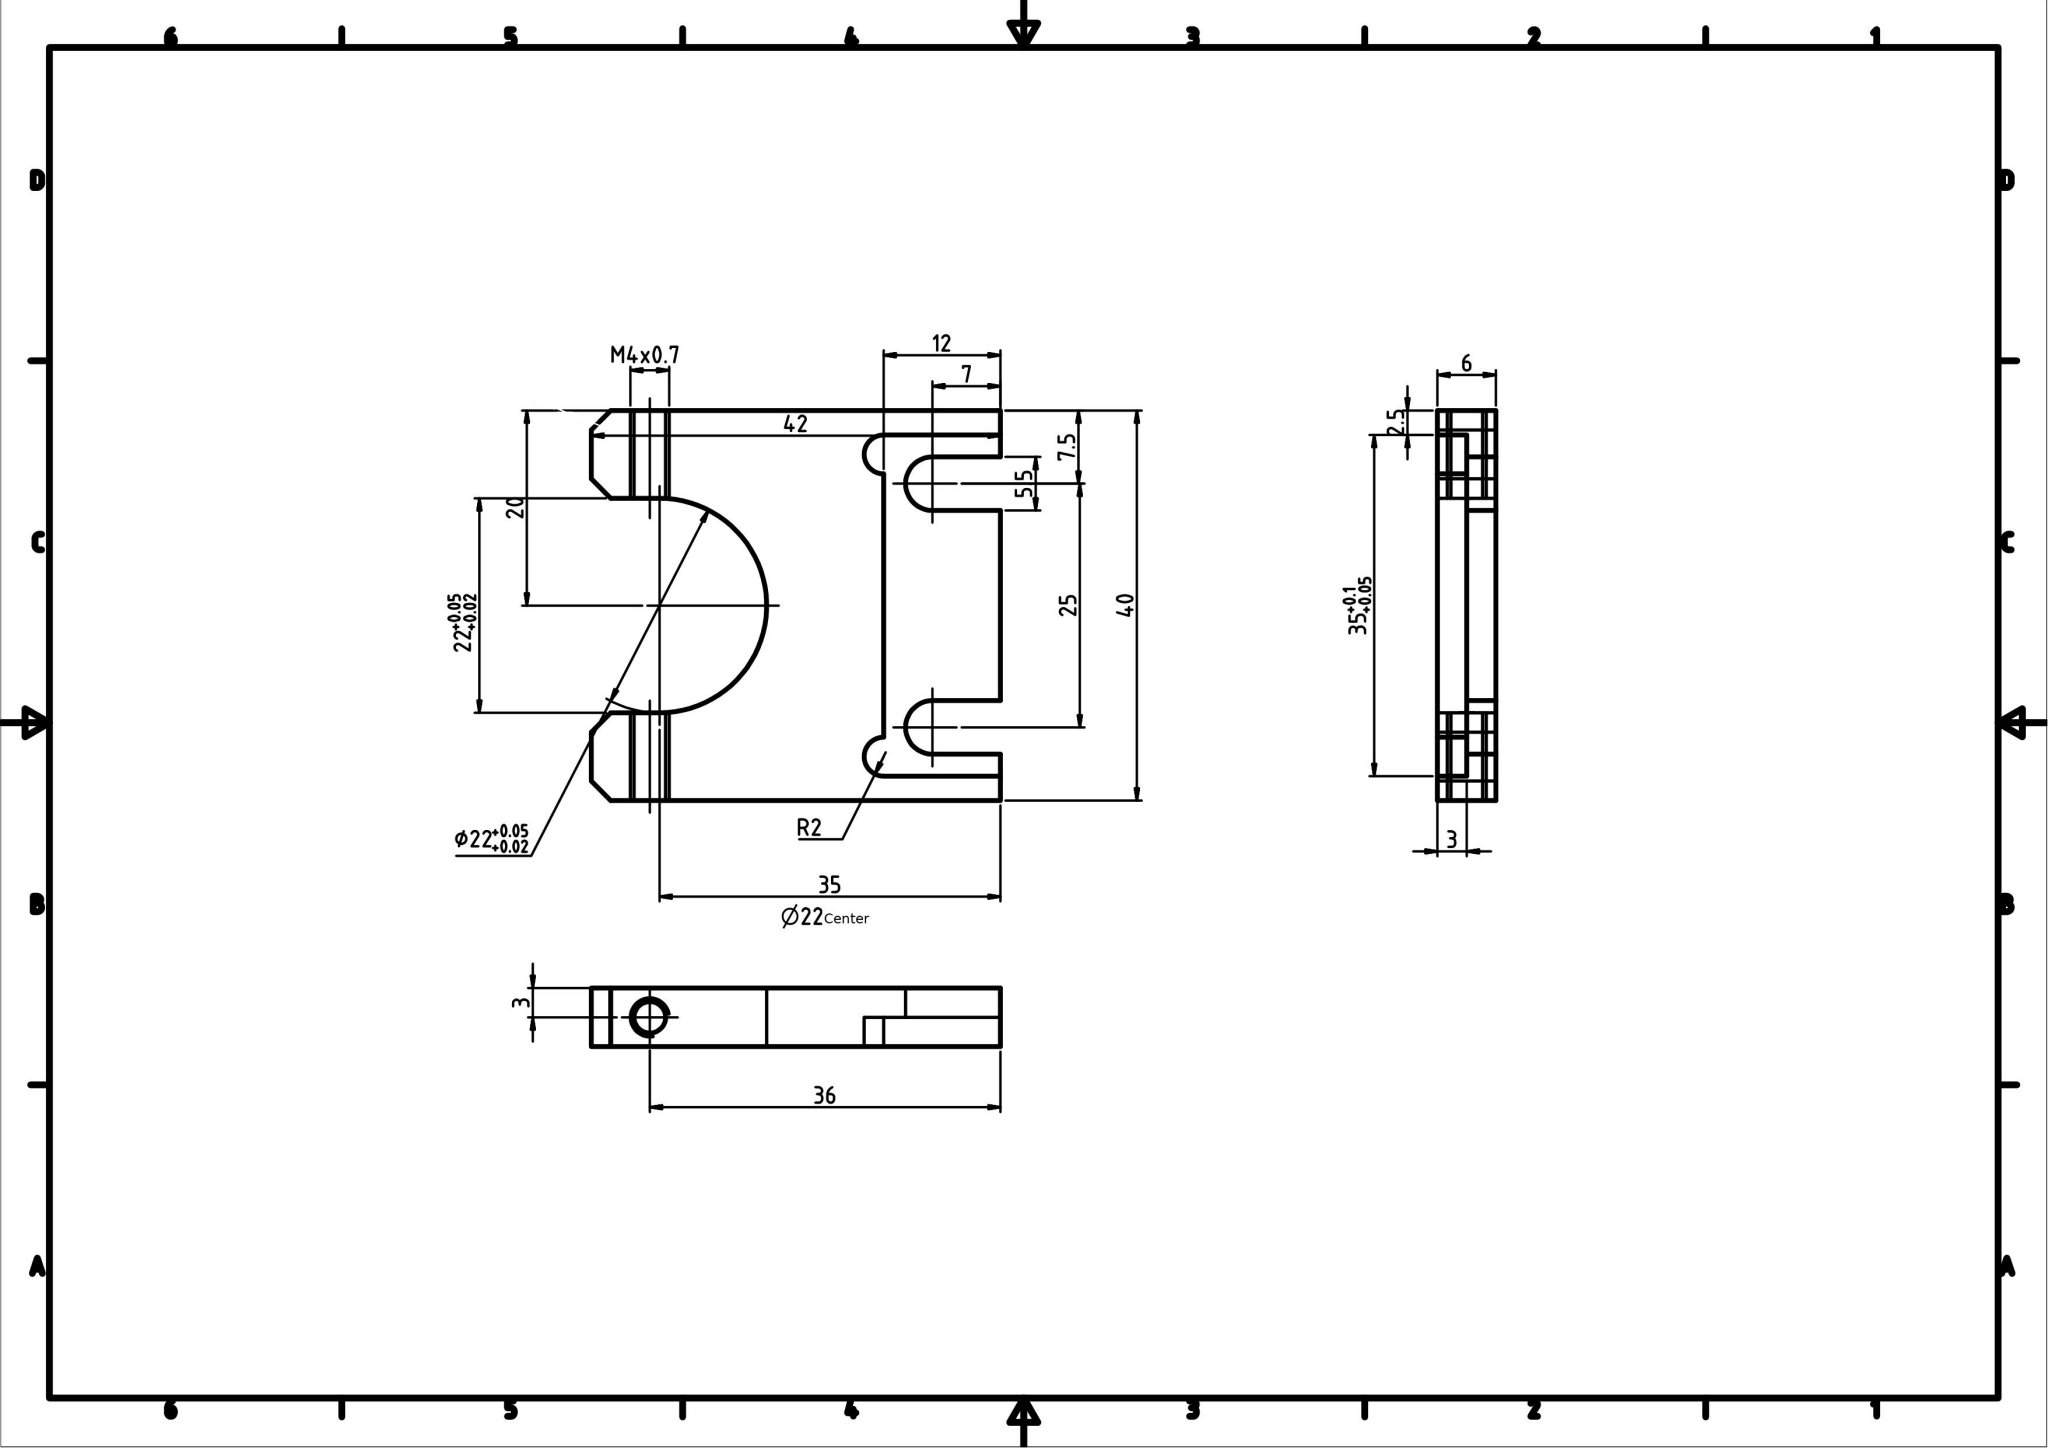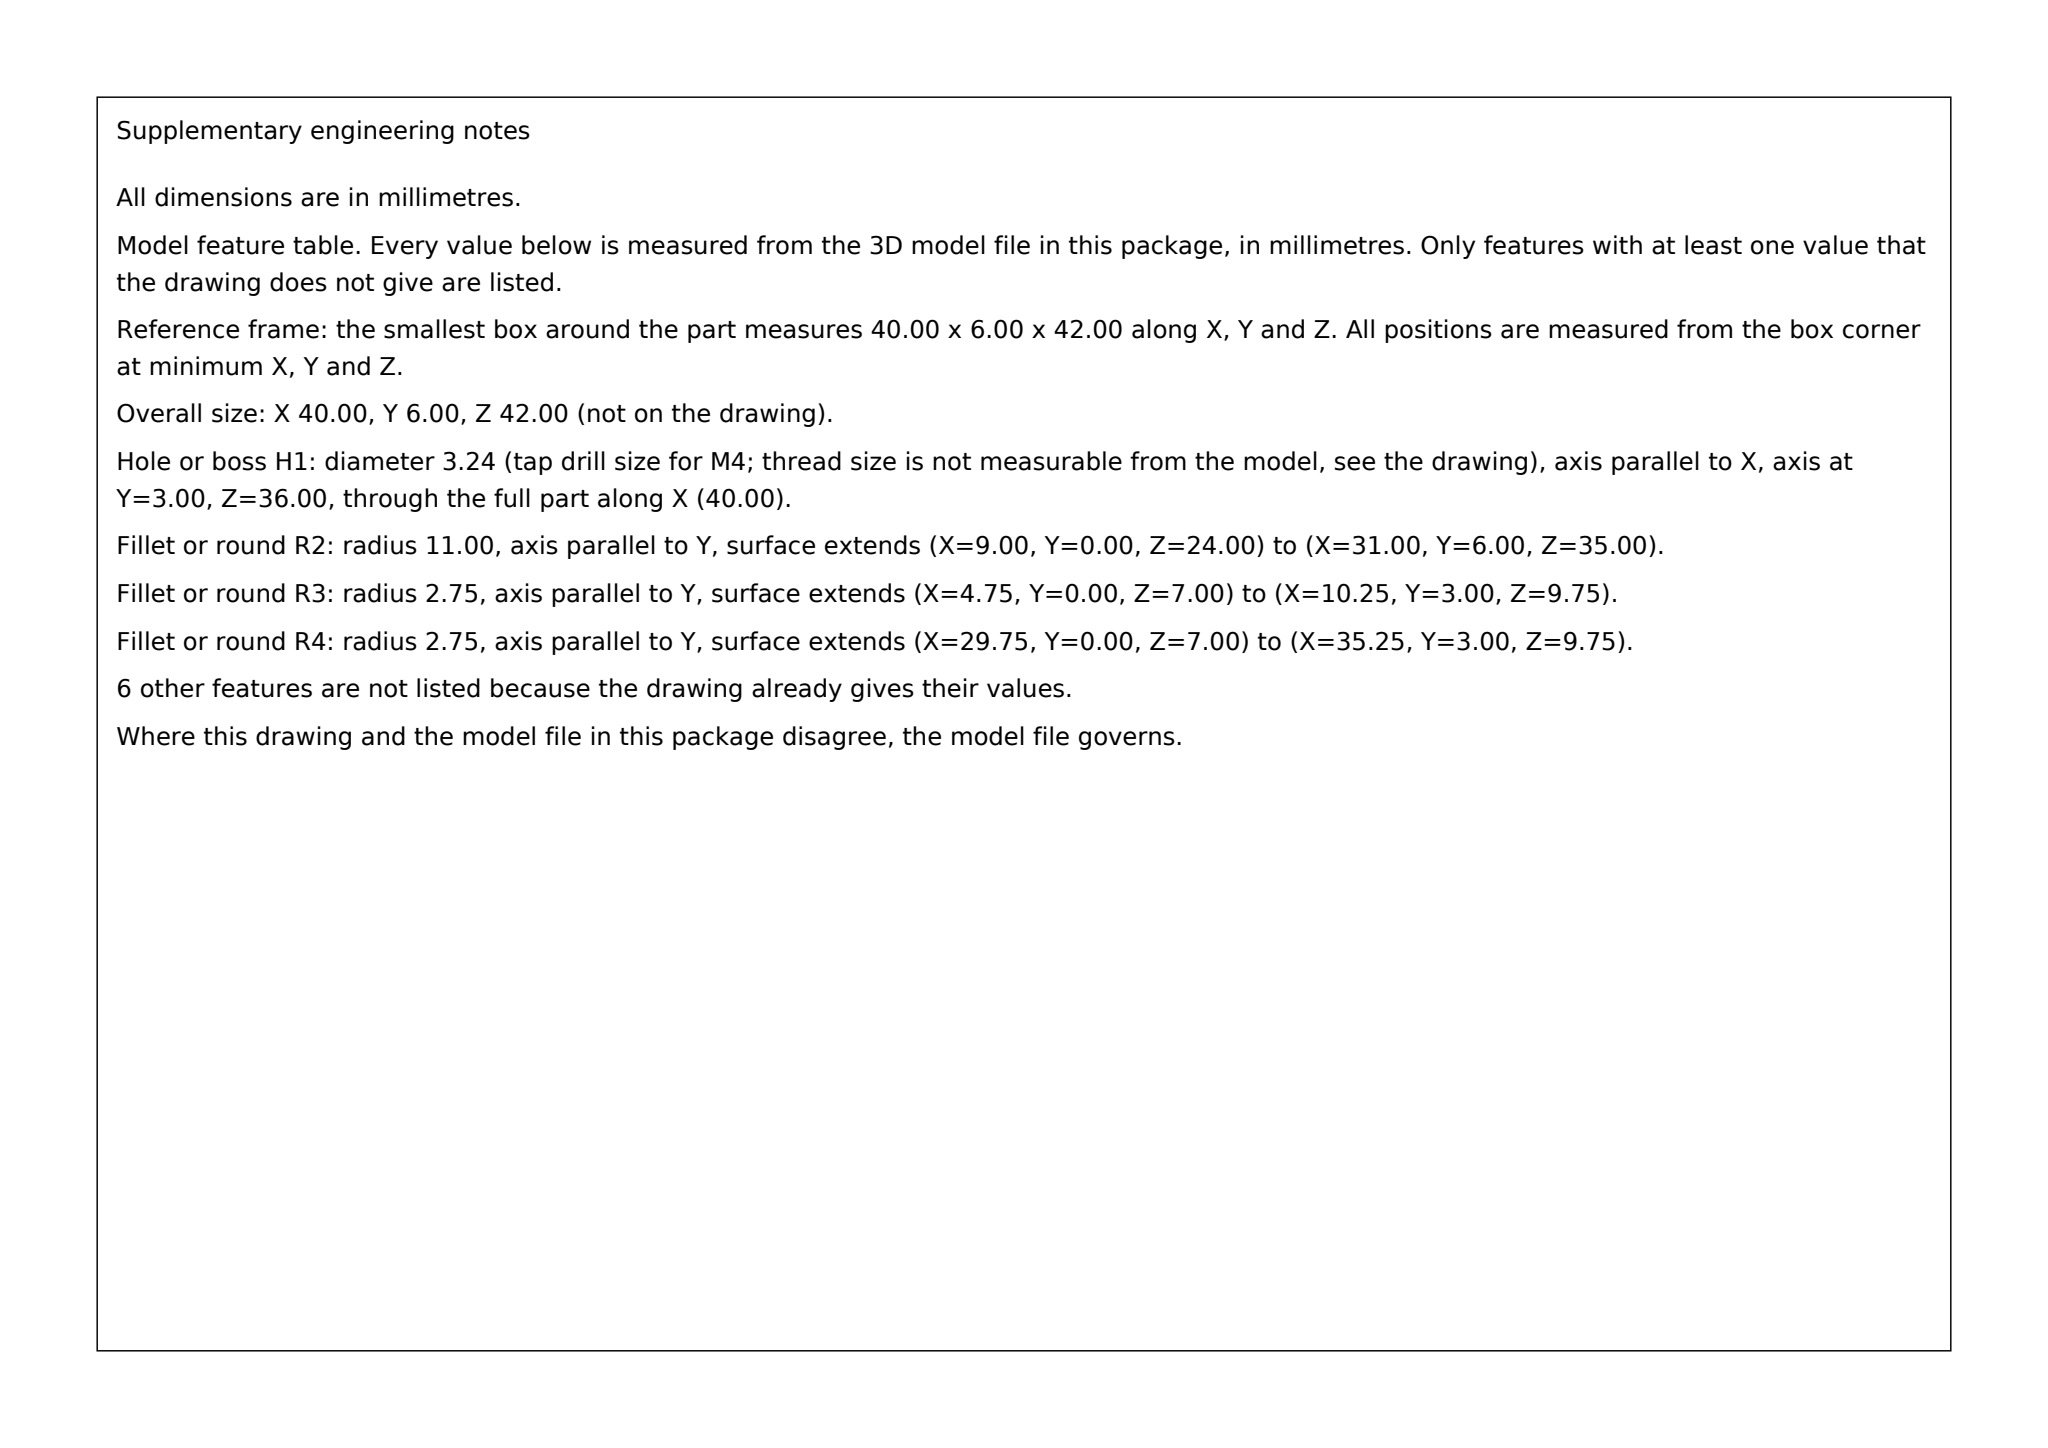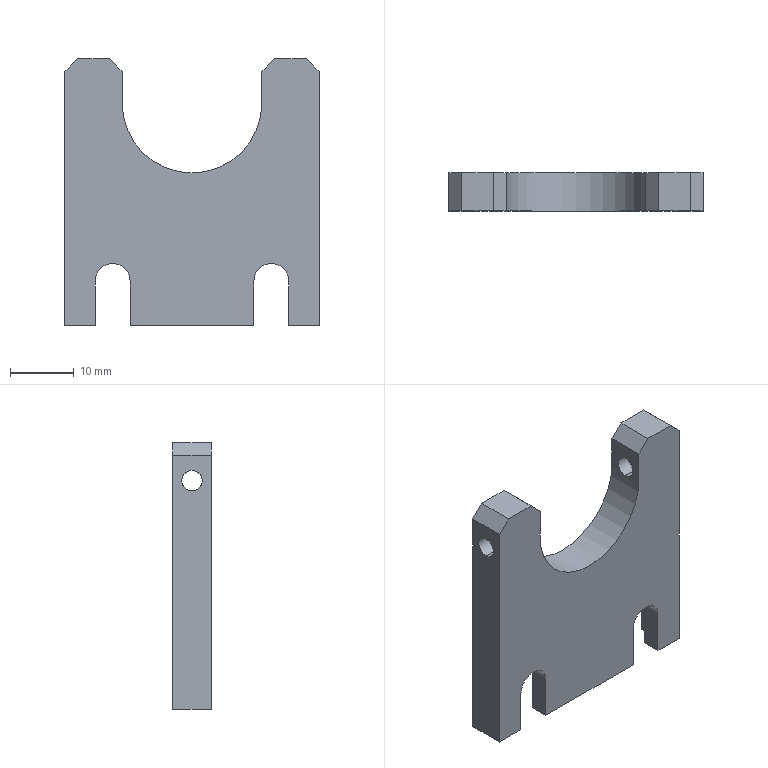Part | SolidWorks | mm | 1 solid | 32 faces | box 40 x 6 x 42 mm | volume 6219 mm3 | plane 23 | cylinder 9 | commonest cylinder face diameters 3.242 x4 4 x2 5.5 x2 22 x1